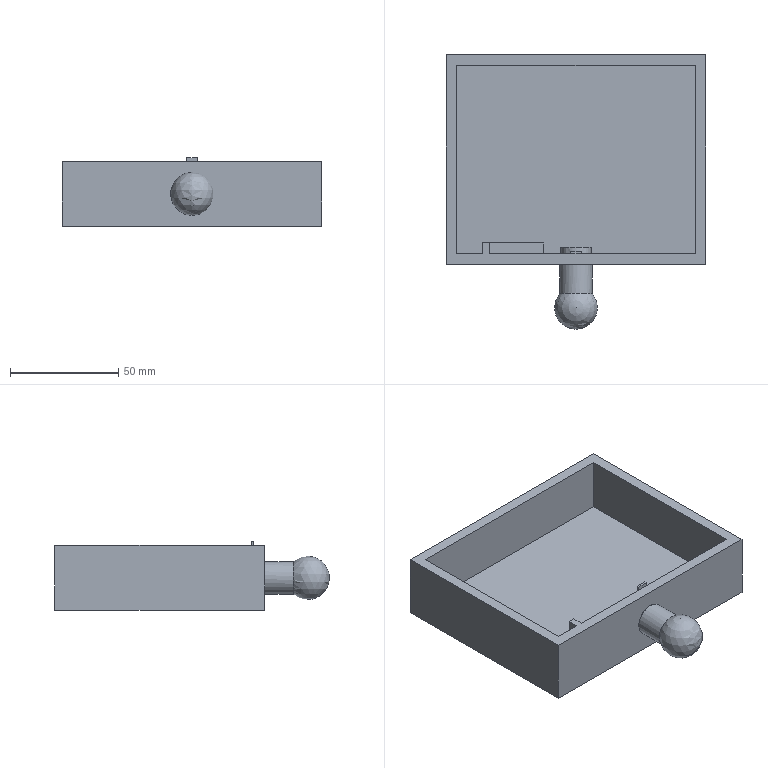Component | NX | SHE_JI-3 | 2 solids | 28 faces | volume 117265 mm3 | plane 24 | cylinder 3 | sphere 1 | commonest cylinder face diameters 15 x2 14 x1